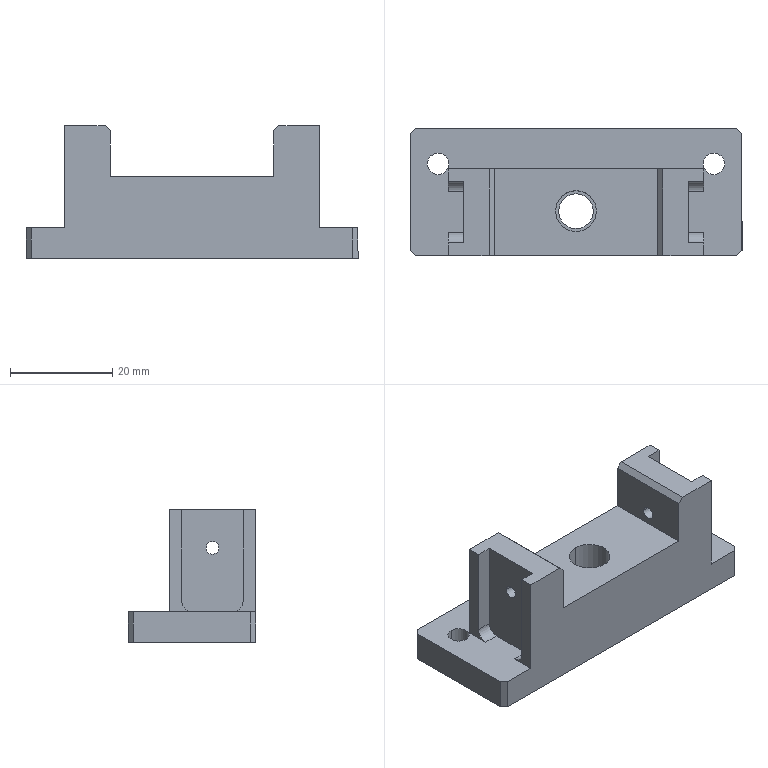Component | SolidWorks | F01AE00111-A2000-21TopEdgeAssembly-1_F01AE00111-A2056-1 | 1 solid | 45 faces | box 65 x 25 x 26 mm | volume 18871 mm3 | plane 29 | cylinder 16 | commonest cylinder face diameters 2.5 x4 4.2 x4 4 x4 8 x2 6.8 x2
build123d program:
from build123d import *

# Parameters (mm, degrees)
BOSS_EXTRUDE1_DEPTH      = 12.5
SKETCH2_W                = 8
SKETCH2_H                = 20
CUT_EXTRUDE1_DEPTH       = 65
M5_TAPPED_HOLE1_D        = 4.2
M5_TAPPED_HOLE1_DEPTH    = 12.4
M5_TAPPED_HOLE1_TIP      = 1.262
SKETCH5_W                = 32
SKETCH5_H                = 10
BOSS_EXTRUDE2_DEPTH      = 17
SKETCH6_W                = 3
SKETCH6_H                = 12
CUT_EXTRUDE2_DEPTH       = 20
M3_TAPPED_HOLE1_D        = 2.5
M3_TAPPED_HOLE1_DEPTH    = 7.5
M3_TAPPED_HOLE1_TIP      = 0.7511
M3_TAPPED_HOLE2_D        = 2.5
M3_TAPPED_HOLE2_DEPTH    = 7.5
M3_TAPPED_HOLE2_TIP      = 0.7511
FILLET1_R                = 2
CHAMFER1_SIZE            = 1
CHAMFER2_SIZE            = 1
M8_TAPPED_HOLE1_D        = 6.8
M8_TAPPED_HOLE1_DEPTH    = 19.75
M8_TAPPED_HOLE1_TIP      = 2.043
SKETCH1_R                = 4
IR_M8_ENGAGEDMAJOR_DEPTH = 6.25


with BuildPart() as part:
    # Sketch1_2 → Boss-Extrude1 (new, symmetric)
    with BuildSketch(Plane.XY):
        Polygon((-32.5, 0), (32.5, 0), (32.5, -6), (25, -6), (25, -26), (16, -26), (16, -6), (-16, -6), (-16, -26), (-25, -26), (-25, -6), (-32.5, -6), align=None)
    extrude(amount=BOSS_EXTRUDE1_DEPTH, both=True)

    # Sketch2 → Cut-Extrude1 (cut)
    with BuildSketch(Plane(origin=(25, 0, 0), x_dir=(0, 0, -1), z_dir=(1, 0, 0))):
        with Locations((-8.5, -16)):
            Rectangle(SKETCH2_W, SKETCH2_H)
    extrude(amount=-CUT_EXTRUDE1_DEPTH, mode=Mode.SUBTRACT)

    # M5 Tapped Hole1
    with Locations(Plane(origin=(0, 0, 0), x_dir=(1, 0, 0), z_dir=(0, 1, 0))):
        with Locations((27, -5.5), (-27, -5.5)):
            Hole(M5_TAPPED_HOLE1_D / 2, depth=M5_TAPPED_HOLE1_DEPTH)
            with Locations((0, 0, -(M5_TAPPED_HOLE1_DEPTH + M5_TAPPED_HOLE1_TIP / 2))):  # 118° drill point
                Cone(0, M5_TAPPED_HOLE1_D / 2, M5_TAPPED_HOLE1_TIP, mode=Mode.SUBTRACT)

    # Sketch5 → Boss-Extrude2 (add)
    with BuildSketch(Plane.XY.offset(4.5)):
        with Locations((0, -11)):
            Rectangle(SKETCH5_W, SKETCH5_H)
    extrude(amount=-BOSS_EXTRUDE2_DEPTH)

    # Sketch6 → Cut-Extrude2 (cut)
    with BuildSketch(Plane.XZ.offset(26)):
        with Locations((23.5, -4)):
            Rectangle(SKETCH6_W, SKETCH6_H)
        with Locations((-23.5, -4)):
            Rectangle(SKETCH6_W, SKETCH6_H)
    extrude(amount=-CUT_EXTRUDE2_DEPTH, mode=Mode.SUBTRACT)

    # M3 Tapped Hole1
    with Locations(Plane(origin=(22, 0, 0), x_dir=(0, 0, -1), z_dir=(1, 0, 0))):
        with Locations((4, -18.5)):
            Hole(M3_TAPPED_HOLE1_D / 2, depth=M3_TAPPED_HOLE1_DEPTH)
            with Locations((0, 0, -(M3_TAPPED_HOLE1_DEPTH + M3_TAPPED_HOLE1_TIP / 2))):  # 118° drill point
                Cone(0, M3_TAPPED_HOLE1_D / 2, M3_TAPPED_HOLE1_TIP, mode=Mode.SUBTRACT)

    # M3 Tapped Hole2
    with Locations(Plane.ZY.offset(22)):
        with Locations((-4, -18.5)):
            Hole(M3_TAPPED_HOLE2_D / 2, depth=M3_TAPPED_HOLE2_DEPTH)
            with Locations((0, 0, -(M3_TAPPED_HOLE2_DEPTH + M3_TAPPED_HOLE2_TIP / 2))):  # 118° drill point
                Cone(0, M3_TAPPED_HOLE2_D / 2, M3_TAPPED_HOLE2_TIP, mode=Mode.SUBTRACT)

    # Fillet1
    fillet1_edges = [part.edges().sort_by_distance(p)[0] for p in [
        (23.5, -6, 2),
        (23.5, -6, -10),
        (-23.5, -6, -10),
        (-23.5, -6, 2),
    ]]
    fillet(fillet1_edges, radius=FILLET1_R)

    # Chamfer1
    chamfer1_edges = [part.edges().sort_by_distance(p)[0] for p in [
        (32.5, -3, -12.5),
        (-32.5, -3, -12.5),
        (32.5, -3, 12.5),
        (-32.5, -3, 12.5),
    ]]
    chamfer(chamfer1_edges, length=CHAMFER1_SIZE)

    # Chamfer2
    chamfer2_edges = [part.edges().sort_by_distance(p)[0] for p in [
        (16, -26, -4),
        (-16, -26, -4),
    ]]
    chamfer(chamfer2_edges, length=CHAMFER2_SIZE)

    # M8 Tapped Hole1
    with Locations(Plane(origin=(0, -16, 0), x_dir=(-1, 0, 0), z_dir=(0, -1, 0))):
        with Locations((0, 3.75)):
            Hole(M8_TAPPED_HOLE1_D / 2, depth=M8_TAPPED_HOLE1_DEPTH)
            with Locations((0, 0, -(M8_TAPPED_HOLE1_DEPTH + M8_TAPPED_HOLE1_TIP / 2))):  # 118° drill point
                Cone(0, M8_TAPPED_HOLE1_D / 2, M8_TAPPED_HOLE1_TIP, mode=Mode.SUBTRACT)

    # Sketch1 → IR_M8_EngagedMajor (cut, symmetric)
    with BuildSketch(Plane(origin=(0, -9.75, 0), x_dir=(1, 0, 0), z_dir=(0, 1, 0))):
        with Locations(Location((0, 3.75, 0), (0, 0, 270))):
            Circle(SKETCH1_R)
    extrude(amount=IR_M8_ENGAGEDMAJOR_DEPTH, both=True, mode=Mode.SUBTRACT)


solid = part.part

# Placed as in the assembly
solid = solid.moved(Location((-109.352, 86.298, -375.975), (-90, 0, 0)))